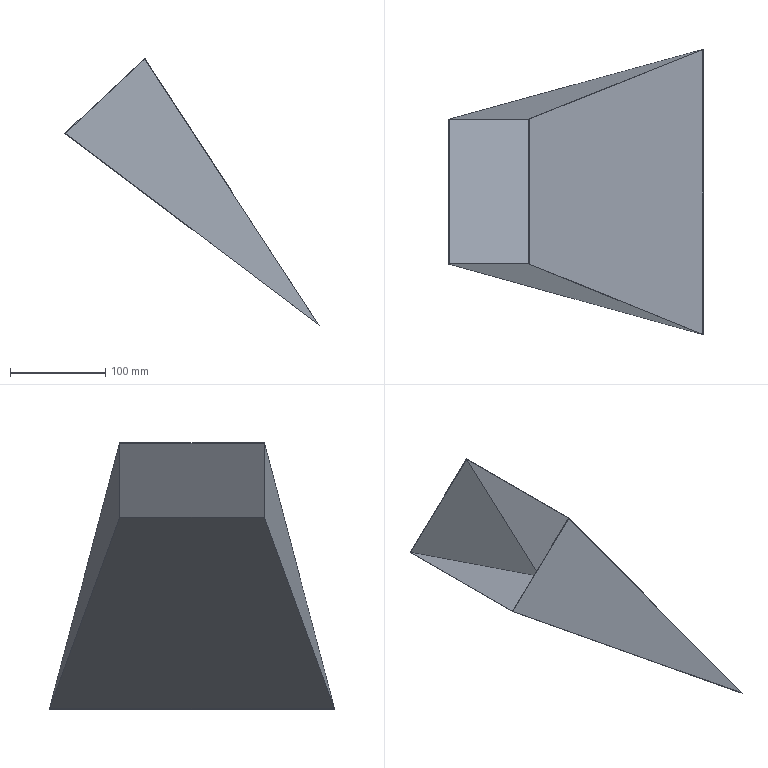Component | SolidWorks | BlowOpenBag-1 | 1 solid | 15 faces | box 267.29 x 300 x 280.4 mm | volume 37906 mm3 | plane 15
build123d program:
from build123d import *

# Parameters (mm, degrees)
BOSS_EXTRUDE1_DEPTH     = 300
CUT_EXTRUDE1_DEPTH      = 450.673
CUT_EXTRUDE1_DEPTH_BACK = 450.673
SHELL1_T                = -0.2
SKETCH3_W               = 114.8
SKETCH3_H               = 151.8
CUT_EXTRUDE2_DEPTH      = 0.5


with BuildPart() as part:
    # Sketch1 → Boss-Extrude1 (new body)
    with BuildSketch(Plane.XY):
        Polygon((0, 0), (57.5, 330), (-57.5, 330), align=None)
    extrude(amount=BOSS_EXTRUDE1_DEPTH)

    # Sketch2 → Cut-Extrude1 (cut, two sides: drawn at the far end of the back side and taken through both)
    with BuildSketch(Plane(origin=(0, 0, 0), x_dir=(0, 0, -1), z_dir=(1, 0, 0)).offset(-CUT_EXTRUDE1_DEPTH_BACK)):
        Polygon((-300, 0), (-226, 330), (-300, 330), align=None)
        Polygon((0, 330), (0, 0), (-74, 330), align=None)
    extrude(amount=CUT_EXTRUDE1_DEPTH + CUT_EXTRUDE1_DEPTH_BACK, mode=Mode.SUBTRACT)

    # Shell1
    shell1_openings = [part.faces().sort_by_distance(p)[0] for p in [
        (0, 330, 150),
    ]]
    offset(amount=SHELL1_T, openings=shell1_openings, kind=Kind.INTERSECTION)

    # Sketch3 → Cut-Extrude2 (cut)
    with BuildSketch(Plane(origin=(0, 330, 0), x_dir=(1, 0, 0), z_dir=(0, 1, 0))):
        with Locations((0, -150)):
            Rectangle(SKETCH3_W, SKETCH3_H)
    extrude(amount=-CUT_EXTRUDE2_DEPTH, mode=Mode.SUBTRACT)


solid = part.part

# Placed as in the assembly
solid = solid.moved(Location((60.974, 109.546, -313.217), (90, 0, 43.049)))
STEP:
#1=COLOUR_RGB('',0.7922,0.8196,0.9333);
#2=FILL_AREA_STYLE_COLOUR('',#1);
#3=FILL_AREA_STYLE('',(#2));
#4=SURFACE_STYLE_FILL_AREA(#3);
#5=SURFACE_SIDE_STYLE('',(#4));
#6=SURFACE_STYLE_USAGE(.BOTH.,#5);
#7=PRESENTATION_STYLE_ASSIGNMENT((#6));
#8=CARTESIAN_POINT('',(-4.817,1.395,-1.295));
#9=VERTEX_POINT('',#8);
#10=CARTESIAN_POINT('',(-8.12,1.395,-4.38));
#11=VERTEX_POINT('',#10);
#12=CARTESIAN_POINT('',(-4.817,1.395,-1.295));
#13=DIRECTION('',(-0.7308,-0.,-0.6826));
#14=VECTOR('',#13,39.37);
#15=LINE('',#12,#14);
#16=EDGE_CURVE('',#9,#11,#15,.T.);
#17=ORIENTED_EDGE('',*,*,#16,.F.);
#18=CARTESIAN_POINT('',(-4.817,-4.581,-1.295));
#19=VERTEX_POINT('',#18);
#20=CARTESIAN_POINT('',(-4.817,-4.581,-1.295));
#21=DIRECTION('',(-0.,1.,-0.));
#22=VECTOR('',#21,39.37);
#23=LINE('',#20,#22);
#24=EDGE_CURVE('',#19,#9,#23,.T.);
#25=ORIENTED_EDGE('',*,*,#24,.F.);
#26=CARTESIAN_POINT('',(-8.12,-4.581,-4.38));
#27=VERTEX_POINT('',#26);
#28=CARTESIAN_POINT('',(-4.817,-4.581,-1.295));
#29=DIRECTION('',(0.7308,0.,0.6826));
#30=VECTOR('',#29,39.37);
#31=LINE('',#28,#30);
#32=EDGE_CURVE('',#27,#19,#31,.T.);
#33=ORIENTED_EDGE('',*,*,#32,.F.);
#34=CARTESIAN_POINT('',(-8.12,-4.581,-4.38));
#35=DIRECTION('',(0.,-1.,0.));
#36=VECTOR('',#35,39.37);
#37=LINE('',#34,#36);
#38=EDGE_CURVE('',#11,#27,#37,.T.);
#39=ORIENTED_EDGE('',*,*,#38,.F.);
#40=EDGE_LOOP('',(#17,#25,#33,#39));
#41=FACE_BOUND('',#40,.T.);
#42=CARTESIAN_POINT('',(-8.123,1.399,-4.383));
#43=VERTEX_POINT('',#42);
#44=CARTESIAN_POINT('',(-8.123,-4.585,-4.383));
#45=VERTEX_POINT('',#44);
#46=CARTESIAN_POINT('',(-8.123,4.313,-4.383));
#47=DIRECTION('',(0.,-1.,0.));
#48=VECTOR('',#47,39.37);
#49=LINE('',#46,#48);
#50=EDGE_CURVE('',#43,#45,#49,.T.);
#51=ORIENTED_EDGE('',*,*,#50,.T.);
#52=CARTESIAN_POINT('',(-4.814,-4.585,-1.292));
#53=VERTEX_POINT('',#52);
#54=CARTESIAN_POINT('',(-4.814,-4.585,-1.292));
#55=DIRECTION('',(-0.7308,-0.,-0.6826));
#56=VECTOR('',#55,39.37);
#57=LINE('',#54,#56);
#58=EDGE_CURVE('',#53,#45,#57,.T.);
#59=ORIENTED_EDGE('',*,*,#58,.F.);
#60=CARTESIAN_POINT('',(-4.814,1.399,-1.292));
#61=VERTEX_POINT('',#60);
#62=CARTESIAN_POINT('',(-4.814,4.313,-1.292));
#63=DIRECTION('',(0.,-1.,0.));
#64=VECTOR('',#63,39.37);
#65=LINE('',#62,#64);
#66=EDGE_CURVE('',#61,#53,#65,.T.);
#67=ORIENTED_EDGE('',*,*,#66,.F.);
#68=CARTESIAN_POINT('',(-4.814,1.399,-1.292));
#69=DIRECTION('',(-0.7308,-0.,-0.6826));
#70=VECTOR('',#69,39.37);
#71=LINE('',#68,#70);
#72=EDGE_CURVE('',#61,#43,#71,.T.);
#73=ORIENTED_EDGE('',*,*,#72,.T.);
#74=EDGE_LOOP('',(#51,#59,#67,#73));
#75=FACE_OUTER_BOUND('',#74,.T.);
#76=CARTESIAN_POINT('',(-4.814,4.313,-1.292));
#77=DIRECTION('',(0.6826,0.,-0.7308));
#78=DIRECTION('',(0.,-1.,0.));
#79=AXIS2_PLACEMENT_3D('',#76,#77,#78);
#80=PLANE('',#79);
#81=ADVANCED_FACE('',(#41,#75),#80,.F.);
#82=ORIENTED_EDGE('',*,*,#66,.T.);
#83=CARTESIAN_POINT('',(2.401,-7.498,-12.331));
#84=VERTEX_POINT('',#83);
#85=CARTESIAN_POINT('',(1.04,-6.949,-10.249));
#86=DIRECTION('',(0.5342,-0.2157,-0.8174));
#87=VECTOR('',#86,39.37);
#88=LINE('',#85,#87);
#89=EDGE_CURVE('',#53,#84,#88,.T.);
#90=ORIENTED_EDGE('',*,*,#89,.T.);
#91=CARTESIAN_POINT('',(2.401,4.313,-12.331));
#92=VERTEX_POINT('',#91);
#93=CARTESIAN_POINT('',(2.401,4.313,-12.331));
#94=DIRECTION('',(0.,-1.,0.));
#95=VECTOR('',#94,39.37);
#96=LINE('',#93,#95);
#97=EDGE_CURVE('',#92,#84,#96,.T.);
#98=ORIENTED_EDGE('',*,*,#97,.F.);
#99=CARTESIAN_POINT('',(2.401,4.313,-12.331));
#100=DIRECTION('',(-0.5342,-0.2157,0.8174));
#101=VECTOR('',#100,39.37);
#102=LINE('',#99,#101);
#103=EDGE_CURVE('',#92,#61,#102,.T.);
#104=ORIENTED_EDGE('',*,*,#103,.T.);
#105=EDGE_LOOP('',(#82,#90,#98,#104));
#106=FACE_OUTER_BOUND('',#105,.T.);
#107=CARTESIAN_POINT('',(2.401,4.313,-12.331));
#108=DIRECTION('',(-0.8371,-0.,-0.5471));
#109=DIRECTION('',(-0.5471,-0.,0.8371));
#110=AXIS2_PLACEMENT_3D('',#107,#108,#109);
#111=PLANE('',#110);
#112=ADVANCED_FACE('',(#106),#111,.F.);
#113=ORIENTED_EDGE('',*,*,#97,.T.);
#114=CARTESIAN_POINT('',(0.4154,-6.949,-10.832));
#115=DIRECTION('',(-0.7792,0.2157,0.5886));
#116=VECTOR('',#115,39.37);
#117=LINE('',#114,#116);
#118=EDGE_CURVE('',#84,#45,#117,.T.);
#119=ORIENTED_EDGE('',*,*,#118,.T.);
#120=ORIENTED_EDGE('',*,*,#50,.F.);
#121=CARTESIAN_POINT('',(2.401,4.313,-12.331));
#122=DIRECTION('',(0.7792,0.2157,-0.5886));
#123=VECTOR('',#122,39.37);
#124=LINE('',#121,#123);
#125=EDGE_CURVE('',#43,#92,#124,.T.);
#126=ORIENTED_EDGE('',*,*,#125,.T.);
#127=EDGE_LOOP('',(#113,#119,#120,#126));
#128=FACE_OUTER_BOUND('',#127,.T.);
#129=CARTESIAN_POINT('',(2.401,4.313,-12.331));
#130=DIRECTION('',(0.6027,0.,0.7979));
#131=DIRECTION('',(0.7979,0.,-0.6027));
#132=AXIS2_PLACEMENT_3D('',#129,#130,#131);
#133=PLANE('',#132);
#134=ADVANCED_FACE('',(#128),#133,.F.);
#135=ORIENTED_EDGE('',*,*,#125,.F.);
#136=ORIENTED_EDGE('',*,*,#72,.F.);
#137=ORIENTED_EDGE('',*,*,#103,.F.);
#138=EDGE_LOOP('',(#135,#136,#137));
#139=FACE_OUTER_BOUND('',#138,.T.);
#140=CARTESIAN_POINT('',(4.055,4.313,-10.786));
#141=DIRECTION('',(0.1494,-0.9758,-0.1599));
#142=DIRECTION('',(-0.6661,-0.2188,0.7131));
#143=AXIS2_PLACEMENT_3D('',#140,#141,#142);
#144=PLANE('',#143);
#145=ADVANCED_FACE('',(#139),#144,.F.);
#146=ORIENTED_EDGE('',*,*,#58,.T.);
#147=ORIENTED_EDGE('',*,*,#118,.F.);
#148=ORIENTED_EDGE('',*,*,#89,.F.);
#149=EDGE_LOOP('',(#146,#147,#148));
#150=FACE_OUTER_BOUND('',#149,.T.);
#151=CARTESIAN_POINT('',(4.055,-7.498,-10.786));
#152=DIRECTION('',(0.1494,0.9758,-0.1599));
#153=DIRECTION('',(0.6661,-0.2188,-0.7131));
#154=AXIS2_PLACEMENT_3D('',#151,#152,#153);
#155=PLANE('',#154);
#156=ADVANCED_FACE('',(#150),#155,.F.);
#157=CARTESIAN_POINT('',(-4.809,-4.581,-1.314));
#158=VERTEX_POINT('',#157);
#159=CARTESIAN_POINT('',(-4.803,-4.581,-1.309));
#160=VERTEX_POINT('',#159);
#161=CARTESIAN_POINT('',(-4.803,-4.581,-1.309));
#162=DIRECTION('',(0.7308,0.,0.6826));
#163=VECTOR('',#162,39.37);
#164=LINE('',#161,#163);
#165=EDGE_CURVE('',#158,#160,#164,.T.);
#166=ORIENTED_EDGE('',*,*,#165,.T.);
#167=CARTESIAN_POINT('',(-4.803,1.395,-1.309));
#168=VERTEX_POINT('',#167);
#169=CARTESIAN_POINT('',(-4.803,-4.581,-1.309));
#170=DIRECTION('',(-0.,1.,-0.));
#171=VECTOR('',#170,39.37);
#172=LINE('',#169,#171);
#173=EDGE_CURVE('',#160,#168,#172,.T.);
#174=ORIENTED_EDGE('',*,*,#173,.T.);
#175=CARTESIAN_POINT('',(-4.809,1.395,-1.314));
#176=VERTEX_POINT('',#175);
#177=CARTESIAN_POINT('',(-4.803,1.395,-1.309));
#178=DIRECTION('',(-0.7308,-0.,-0.6826));
#179=VECTOR('',#178,39.37);
#180=LINE('',#177,#179);
#181=EDGE_CURVE('',#168,#176,#180,.T.);
#182=ORIENTED_EDGE('',*,*,#181,.T.);
#183=CARTESIAN_POINT('',(-4.809,4.313,-1.314));
#184=DIRECTION('',(-0.,1.,-0.));
#185=VECTOR('',#184,39.37);
#186=LINE('',#183,#185);
#187=EDGE_CURVE('',#158,#176,#186,.T.);
#188=ORIENTED_EDGE('',*,*,#187,.F.);
#189=EDGE_LOOP('',(#166,#174,#182,#188));
#190=FACE_OUTER_BOUND('',#189,.T.);
#191=CARTESIAN_POINT('',(-6.455,-7.498,-2.852));
#192=DIRECTION('',(-0.6826,-0.,0.7308));
#193=DIRECTION('',(-0.,1.,-0.));
#194=AXIS2_PLACEMENT_3D('',#191,#192,#193);
#195=PLANE('',#194);
#196=ADVANCED_FACE('',(#190),#195,.T.);
#197=ORIENTED_EDGE('',*,*,#24,.T.);
#198=CARTESIAN_POINT('',(-4.803,1.395,-1.309));
#199=DIRECTION('',(-0.6826,-0.,0.7308));
#200=VECTOR('',#199,39.37);
#201=LINE('',#198,#200);
#202=EDGE_CURVE('',#168,#9,#201,.T.);
#203=ORIENTED_EDGE('',*,*,#202,.F.);
#204=ORIENTED_EDGE('',*,*,#173,.F.);
#205=CARTESIAN_POINT('',(-4.803,-4.581,-1.309));
#206=DIRECTION('',(-0.6826,-0.,0.7308));
#207=VECTOR('',#206,39.37);
#208=LINE('',#205,#207);
#209=EDGE_CURVE('',#160,#19,#208,.T.);
#210=ORIENTED_EDGE('',*,*,#209,.T.);
#211=EDGE_LOOP('',(#197,#203,#204,#210));
#212=FACE_OUTER_BOUND('',#211,.T.);
#213=CARTESIAN_POINT('',(-4.803,-4.581,-1.309));
#214=DIRECTION('',(0.7308,0.,0.6826));
#215=DIRECTION('',(-0.,1.,-0.));
#216=AXIS2_PLACEMENT_3D('',#213,#214,#215);
#217=PLANE('',#216);
#218=ADVANCED_FACE('',(#212),#217,.F.);
#219=CARTESIAN_POINT('',(-4.81,-4.581,-1.313));
#220=VERTEX_POINT('',#219);
#221=CARTESIAN_POINT('',(2.394,-4.581,-12.336));
#222=DIRECTION('',(-0.5471,-0.,0.8371));
#223=VECTOR('',#222,39.37);
#224=LINE('',#221,#223);
#225=EDGE_CURVE('',#158,#220,#224,.T.);
#226=ORIENTED_EDGE('',*,*,#225,.T.);
#227=CARTESIAN_POINT('',(-8.102,-4.581,-4.388));
#228=VERTEX_POINT('',#227);
#229=CARTESIAN_POINT('',(-4.801,-4.581,-1.305));
#230=DIRECTION('',(-0.7308,-0.,-0.6826));
#231=VECTOR('',#230,39.37);
#232=LINE('',#229,#231);
#233=EDGE_CURVE('',#220,#228,#232,.T.);
#234=ORIENTED_EDGE('',*,*,#233,.T.);
#235=CARTESIAN_POINT('',(-8.101,-4.581,-4.389));
#236=VERTEX_POINT('',#235);
#237=CARTESIAN_POINT('',(2.405,-4.581,-12.325));
#238=DIRECTION('',(0.7979,0.,-0.6027));
#239=VECTOR('',#238,39.37);
#240=LINE('',#237,#239);
#241=EDGE_CURVE('',#228,#236,#240,.T.);
#242=ORIENTED_EDGE('',*,*,#241,.T.);
#243=CARTESIAN_POINT('',(-8.106,-4.581,-4.394));
#244=VERTEX_POINT('',#243);
#245=CARTESIAN_POINT('',(-4.803,-4.581,-1.309));
#246=DIRECTION('',(0.7308,0.,0.6826));
#247=VECTOR('',#246,39.37);
#248=LINE('',#245,#247);
#249=EDGE_CURVE('',#244,#236,#248,.T.);
#250=ORIENTED_EDGE('',*,*,#249,.F.);
#251=CARTESIAN_POINT('',(-8.106,-4.581,-4.394));
#252=DIRECTION('',(-0.6826,-0.,0.7308));
#253=VECTOR('',#252,39.37);
#254=LINE('',#251,#253);
#255=EDGE_CURVE('',#244,#27,#254,.T.);
#256=ORIENTED_EDGE('',*,*,#255,.T.);
#257=ORIENTED_EDGE('',*,*,#32,.T.);
#258=ORIENTED_EDGE('',*,*,#209,.F.);
#259=ORIENTED_EDGE('',*,*,#165,.F.);
#260=EDGE_LOOP('',(#226,#234,#242,#250,#256,#257,#258,#259));
#261=FACE_OUTER_BOUND('',#260,.T.);
#262=CARTESIAN_POINT('',(-4.803,-4.581,-1.309));
#263=DIRECTION('',(0.,-1.,0.));
#264=DIRECTION('',(0.7308,0.,0.6826));
#265=AXIS2_PLACEMENT_3D('',#262,#263,#264);
#266=PLANE('',#265);
#267=ADVANCED_FACE('',(#261),#266,.F.);
#268=ORIENTED_EDGE('',*,*,#38,.T.);
#269=ORIENTED_EDGE('',*,*,#255,.F.);
#270=CARTESIAN_POINT('',(-8.106,1.395,-4.394));
#271=VERTEX_POINT('',#270);
#272=CARTESIAN_POINT('',(-8.106,-4.581,-4.394));
#273=DIRECTION('',(0.,-1.,0.));
#274=VECTOR('',#273,39.37);
#275=LINE('',#272,#274);
#276=EDGE_CURVE('',#271,#244,#275,.T.);
#277=ORIENTED_EDGE('',*,*,#276,.F.);
#278=CARTESIAN_POINT('',(-8.106,1.395,-4.394));
#279=DIRECTION('',(-0.6826,-0.,0.7308));
#280=VECTOR('',#279,39.37);
#281=LINE('',#278,#280);
#282=EDGE_CURVE('',#271,#11,#281,.T.);
#283=ORIENTED_EDGE('',*,*,#282,.T.);
#284=EDGE_LOOP('',(#268,#269,#277,#283));
#285=FACE_OUTER_BOUND('',#284,.T.);
#286=CARTESIAN_POINT('',(-8.106,-4.581,-4.394));
#287=DIRECTION('',(-0.7308,-0.,-0.6826));
#288=DIRECTION('',(0.,-1.,0.));
#289=AXIS2_PLACEMENT_3D('',#286,#287,#288);
#290=PLANE('',#289);
#291=ADVANCED_FACE('',(#285),#290,.F.);
#292=CARTESIAN_POINT('',(-4.81,1.395,-1.313));
#293=VERTEX_POINT('',#292);
#294=CARTESIAN_POINT('',(2.394,1.395,-12.336));
#295=DIRECTION('',(0.5471,0.,-0.8371));
#296=VECTOR('',#295,39.37);
#297=LINE('',#294,#296);
#298=EDGE_CURVE('',#293,#176,#297,.T.);
#299=ORIENTED_EDGE('',*,*,#298,.T.);
#300=ORIENTED_EDGE('',*,*,#181,.F.);
#301=ORIENTED_EDGE('',*,*,#202,.T.);
#302=ORIENTED_EDGE('',*,*,#16,.T.);
#303=ORIENTED_EDGE('',*,*,#282,.F.);
#304=CARTESIAN_POINT('',(-8.101,1.395,-4.389));
#305=VERTEX_POINT('',#304);
#306=CARTESIAN_POINT('',(-4.803,1.395,-1.309));
#307=DIRECTION('',(-0.7308,-0.,-0.6826));
#308=VECTOR('',#307,39.37);
#309=LINE('',#306,#308);
#310=EDGE_CURVE('',#305,#271,#309,.T.);
#311=ORIENTED_EDGE('',*,*,#310,.F.);
#312=CARTESIAN_POINT('',(-8.102,1.395,-4.388));
#313=VERTEX_POINT('',#312);
#314=CARTESIAN_POINT('',(2.405,1.395,-12.325));
#315=DIRECTION('',(-0.7979,-0.,0.6027));
#316=VECTOR('',#315,39.37);
#317=LINE('',#314,#316);
#318=EDGE_CURVE('',#305,#313,#317,.T.);
#319=ORIENTED_EDGE('',*,*,#318,.T.);
#320=CARTESIAN_POINT('',(-4.801,1.395,-1.305));
#321=DIRECTION('',(0.7308,0.,0.6826));
#322=VECTOR('',#321,39.37);
#323=LINE('',#320,#322);
#324=EDGE_CURVE('',#313,#293,#323,.T.);
#325=ORIENTED_EDGE('',*,*,#324,.T.);
#326=EDGE_LOOP('',(#299,#300,#301,#302,#303,#311,#319,#325));
#327=FACE_OUTER_BOUND('',#326,.T.);
#328=CARTESIAN_POINT('',(-4.803,1.395,-1.309));
#329=DIRECTION('',(-0.,1.,-0.));
#330=DIRECTION('',(-0.7308,-0.,-0.6826));
#331=AXIS2_PLACEMENT_3D('',#328,#329,#330);
#332=PLANE('',#331);
#333=ADVANCED_FACE('',(#327),#332,.F.);
#334=ORIENTED_EDGE('',*,*,#310,.T.);
#335=ORIENTED_EDGE('',*,*,#276,.T.);
#336=ORIENTED_EDGE('',*,*,#249,.T.);
#337=CARTESIAN_POINT('',(-8.101,4.313,-4.389));
#338=DIRECTION('',(0.,-1.,0.));
#339=VECTOR('',#338,39.37);
#340=LINE('',#337,#339);
#341=EDGE_CURVE('',#305,#236,#340,.T.);
#342=ORIENTED_EDGE('',*,*,#341,.F.);
#343=EDGE_LOOP('',(#334,#335,#336,#342));
#344=FACE_OUTER_BOUND('',#343,.T.);
#345=CARTESIAN_POINT('',(-6.455,-7.498,-2.852));
#346=DIRECTION('',(-0.6826,-0.,0.7308));
#347=DIRECTION('',(-0.,1.,-0.));
#348=AXIS2_PLACEMENT_3D('',#345,#346,#347);
#349=PLANE('',#348);
#350=ADVANCED_FACE('',(#344),#349,.T.);
#351=ORIENTED_EDGE('',*,*,#324,.F.);
#352=CARTESIAN_POINT('',(2.369,4.294,-12.298));
#353=VERTEX_POINT('',#352);
#354=CARTESIAN_POINT('',(2.407,4.305,-12.326));
#355=DIRECTION('',(0.7792,0.2157,-0.5886));
#356=VECTOR('',#355,39.37);
#357=LINE('',#354,#356);
#358=EDGE_CURVE('',#313,#353,#357,.T.);
#359=ORIENTED_EDGE('',*,*,#358,.T.);
#360=CARTESIAN_POINT('',(2.395,4.305,-12.337));
#361=DIRECTION('',(-0.5342,-0.2157,0.8174));
#362=VECTOR('',#361,39.37);
#363=LINE('',#360,#362);
#364=EDGE_CURVE('',#353,#293,#363,.T.);
#365=ORIENTED_EDGE('',*,*,#364,.T.);
#366=EDGE_LOOP('',(#351,#359,#365));
#367=FACE_OUTER_BOUND('',#366,.T.);
#368=CARTESIAN_POINT('',(4.056,4.305,-10.787));
#369=DIRECTION('',(0.1494,-0.9758,-0.1599));
#370=DIRECTION('',(-0.6661,-0.2188,0.7131));
#371=AXIS2_PLACEMENT_3D('',#368,#369,#370);
#372=PLANE('',#371);
#373=ADVANCED_FACE('',(#367),#372,.T.);
#374=ORIENTED_EDGE('',*,*,#233,.F.);
#375=CARTESIAN_POINT('',(2.369,-7.48,-12.298));
#376=VERTEX_POINT('',#375);
#377=CARTESIAN_POINT('',(1.034,-6.941,-10.255));
#378=DIRECTION('',(0.5342,-0.2157,-0.8174));
#379=VECTOR('',#378,39.37);
#380=LINE('',#377,#379);
#381=EDGE_CURVE('',#220,#376,#380,.T.);
#382=ORIENTED_EDGE('',*,*,#381,.T.);
#383=CARTESIAN_POINT('',(0.4216,-6.941,-10.827));
#384=DIRECTION('',(-0.7792,0.2157,0.5886));
#385=VECTOR('',#384,39.37);
#386=LINE('',#383,#385);
#387=EDGE_CURVE('',#376,#228,#386,.T.);
#388=ORIENTED_EDGE('',*,*,#387,.T.);
#389=EDGE_LOOP('',(#374,#382,#388));
#390=FACE_OUTER_BOUND('',#389,.T.);
#391=CARTESIAN_POINT('',(4.056,-7.491,-10.787));
#392=DIRECTION('',(0.1494,0.9758,-0.1599));
#393=DIRECTION('',(0.6661,-0.2188,-0.7131));
#394=AXIS2_PLACEMENT_3D('',#391,#392,#393);
#395=PLANE('',#394);
#396=ADVANCED_FACE('',(#390),#395,.T.);
#397=ORIENTED_EDGE('',*,*,#241,.F.);
#398=ORIENTED_EDGE('',*,*,#387,.F.);
#399=CARTESIAN_POINT('',(2.369,4.313,-12.298));
#400=DIRECTION('',(0.,-1.,0.));
#401=VECTOR('',#400,39.37);
#402=LINE('',#399,#401);
#403=EDGE_CURVE('',#353,#376,#402,.T.);
#404=ORIENTED_EDGE('',*,*,#403,.F.);
#405=ORIENTED_EDGE('',*,*,#358,.F.);
#406=ORIENTED_EDGE('',*,*,#318,.F.);
#407=ORIENTED_EDGE('',*,*,#341,.T.);
#408=EDGE_LOOP('',(#397,#398,#404,#405,#406,#407));
#409=FACE_OUTER_BOUND('',#408,.T.);
#410=CARTESIAN_POINT('',(2.405,4.313,-12.325));
#411=DIRECTION('',(0.6027,0.,0.7979));
#412=DIRECTION('',(0.7979,0.,-0.6027));
#413=AXIS2_PLACEMENT_3D('',#410,#411,#412);
#414=PLANE('',#413);
#415=ADVANCED_FACE('',(#409),#414,.T.);
#416=ORIENTED_EDGE('',*,*,#225,.F.);
#417=ORIENTED_EDGE('',*,*,#187,.T.);
#418=ORIENTED_EDGE('',*,*,#298,.F.);
#419=ORIENTED_EDGE('',*,*,#364,.F.);
#420=ORIENTED_EDGE('',*,*,#403,.T.);
#421=ORIENTED_EDGE('',*,*,#381,.F.);
#422=EDGE_LOOP('',(#416,#417,#418,#419,#420,#421));
#423=FACE_OUTER_BOUND('',#422,.T.);
#424=CARTESIAN_POINT('',(2.394,4.313,-12.336));
#425=DIRECTION('',(-0.8371,-0.,-0.5471));
#426=DIRECTION('',(-0.5471,-0.,0.8371));
#427=AXIS2_PLACEMENT_3D('',#424,#425,#426);
#428=PLANE('',#427);
#429=ADVANCED_FACE('',(#423),#428,.T.);
#430=CLOSED_SHELL('',(#81,#112,#134,#145,#156,#196,#218,#267,#291,#333,#350,#373,#396,#415,#429));
#431=MANIFOLD_SOLID_BREP('',#430);
#432=STYLED_ITEM('',(#7),#431);
#433=PRESENTATION_LAYER_ASSIGNMENT('','',(#432));
#434=(LENGTH_UNIT()NAMED_UNIT(*)SI_UNIT($,.METRE.));
#435=LENGTH_MEASURE_WITH_UNIT(LENGTH_MEASURE(0.0254),#434);
#436=DIMENSIONAL_EXPONENTS(1.,0.,0.,0.,0.,0.,0.);
#437=(CONVERSION_BASED_UNIT('',#435)LENGTH_UNIT()NAMED_UNIT(#436));
#438=UNCERTAINTY_MEASURE_WITH_UNIT(LENGTH_MEASURE(0.00001),#437,'','');
#439=(NAMED_UNIT(*)PLANE_ANGLE_UNIT()SI_UNIT($,.RADIAN.));
#440=(NAMED_UNIT(*)SI_UNIT($,.STERADIAN.)SOLID_ANGLE_UNIT());
#441=(GEOMETRIC_REPRESENTATION_CONTEXT(3)GLOBAL_UNCERTAINTY_ASSIGNED_CONTEXT((#438))GLOBAL_UNIT_ASSIGNED_CONTEXT((#437,#439,#440))REPRESENTATION_CONTEXT('',''));
#442=MECHANICAL_DESIGN_GEOMETRIC_PRESENTATION_REPRESENTATION('',(#432),#441);
#443=CARTESIAN_POINT('',(0.,0.,0.));
#444=DIRECTION('',(0.,0.,1.));
#445=DIRECTION('',(1.,0.,0.));
#446=AXIS2_PLACEMENT_3D('',#443,#444,#445);
#447=(LENGTH_UNIT()NAMED_UNIT(*)SI_UNIT($,.METRE.));
#448=LENGTH_MEASURE_WITH_UNIT(LENGTH_MEASURE(0.0254),#447);
#449=DIMENSIONAL_EXPONENTS(1.,0.,0.,0.,0.,0.,0.);
#450=(CONVERSION_BASED_UNIT('',#448)LENGTH_UNIT()NAMED_UNIT(#449));
#451=UNCERTAINTY_MEASURE_WITH_UNIT(LENGTH_MEASURE(0.00001),#450,'','');
#452=(NAMED_UNIT(*)PLANE_ANGLE_UNIT()SI_UNIT($,.RADIAN.));
#453=(NAMED_UNIT(*)SI_UNIT($,.STERADIAN.)SOLID_ANGLE_UNIT());
#454=(GEOMETRIC_REPRESENTATION_CONTEXT(3)GLOBAL_UNCERTAINTY_ASSIGNED_CONTEXT((#451))GLOBAL_UNIT_ASSIGNED_CONTEXT((#450,#452,#453))REPRESENTATION_CONTEXT('',''));
#455=ADVANCED_BREP_SHAPE_REPRESENTATION('',(#431,#446),#454);